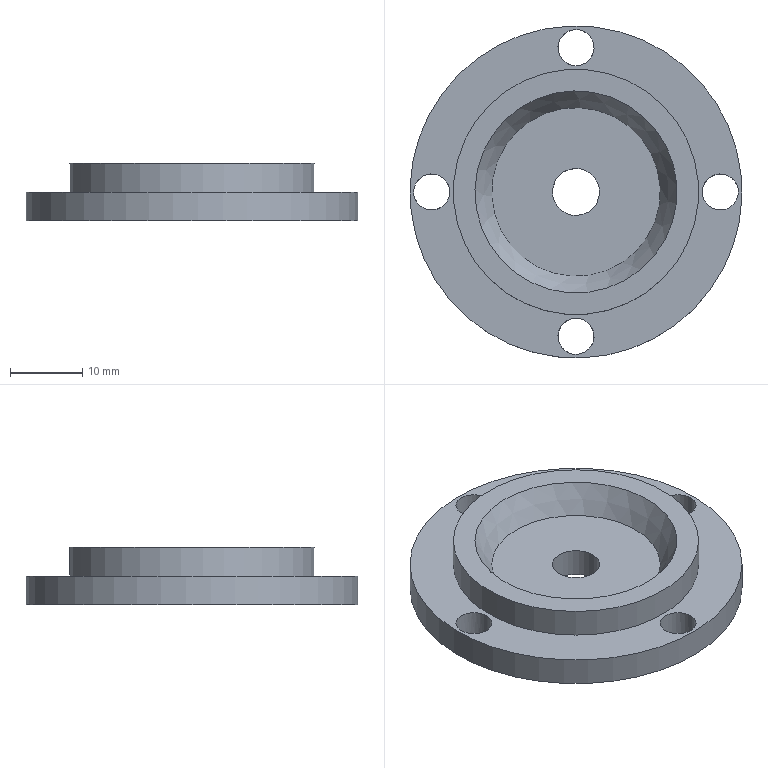Component | NX | BEARING_COVER | 1 solid | 12 faces | box 46 x 46 x 8 mm | volume 7753 mm3 | cylinder 7 | plane 4 | cone 1 | commonest cylinder face diameters 5 x4 46 x1 34 x1 6.5 x1
STEP:
#1=CARTESIAN_POINT('',(0.,0.,0.));
#2=DIRECTION('',(0.,0.,1.));
#3=DIRECTION('',(1.,0.,0.));
#4=AXIS2_PLACEMENT_3D('',#1,#2,#3);
#5=CARTESIAN_POINT('',(609.426,-134.038,-1192.));
#6=VERTEX_POINT('',#5);
#7=CARTESIAN_POINT('',(625.689,-150.302,-1192.));
#8=DIRECTION('',(0.,0.,1.));
#9=DIRECTION('',(-0.7071,0.7071,0.));
#10=AXIS2_PLACEMENT_3D('',#7,#8,#9);
#11=CIRCLE('',#10,23.);
#12=CARTESIAN_POINT('',(625.689,-150.302,-1188.));
#13=DIRECTION('',(0.,0.,1.));
#14=DIRECTION('',(-0.7071,0.7071,0.));
#15=AXIS2_PLACEMENT_3D('',#12,#13,#14);
#16=CYLINDRICAL_SURFACE('',#15,23.);
#17=CARTESIAN_POINT('',(0.,-4.));
#18=DIRECTION('',(1.,0.));
#19=VECTOR('',#18,1.);
#20=LINE('',#17,#19);
#21=(GEOMETRIC_REPRESENTATION_CONTEXT(2)PARAMETRIC_REPRESENTATION_CONTEXT()REPRESENTATION_CONTEXT('',''));
#22=DEFINITIONAL_REPRESENTATION('',(#20),#21);
#23=PCURVE('',#16,#22);
#24=CARTESIAN_POINT('',(641.952,-134.038,-1192.));
#25=DIRECTION('',(0.,0.,-1.));
#26=DIRECTION('',(0.7071,-0.7071,0.));
#27=AXIS2_PLACEMENT_3D('',#24,#25,#26);
#28=PLANE('',#27);
#29=CARTESIAN_POINT('',(-23.,23.));
#30=CARTESIAN_POINT('',(-23.,62.837));
#31=CARTESIAN_POINT('',(11.5,42.919));
#32=CARTESIAN_POINT('',(46.,23.));
#33=CARTESIAN_POINT('',(11.5,3.081));
#34=CARTESIAN_POINT('',(-23.,-16.837));
#35=CARTESIAN_POINT('',(-23.,23.));
#36=(BOUNDED_CURVE()B_SPLINE_CURVE(2,(#29,#30,#31,#32,#33,#34,#35),.UNSPECIFIED.,.T.,.F.)B_SPLINE_CURVE_WITH_KNOTS((1,2,2,2,2,1),(-2.094,0.,2.094,4.189,6.283,8.378),.UNSPECIFIED.)CURVE()GEOMETRIC_REPRESENTATION_ITEM()RATIONAL_B_SPLINE_CURVE((1.,0.5,1.,0.5,1.,0.5,1.))REPRESENTATION_ITEM(''));
#37=(GEOMETRIC_REPRESENTATION_CONTEXT(2)PARAMETRIC_REPRESENTATION_CONTEXT()REPRESENTATION_CONTEXT('',''));
#38=DEFINITIONAL_REPRESENTATION('',(#36),#37);
#39=PCURVE('',#28,#38);
#40=SURFACE_CURVE('',#11,(#23,#39),.PCURVE_S1.);
#41=EDGE_CURVE('',#6,#6,#40,.T.);
#42=ORIENTED_EDGE('',*,*,#41,.F.);
#43=CARTESIAN_POINT('',(609.426,-134.038,-1196.));
#44=VERTEX_POINT('',#43);
#45=CARTESIAN_POINT('',(609.426,-134.038,-1196.));
#46=CARTESIAN_POINT('',(609.426,-134.038,-1192.));
#47=B_SPLINE_CURVE_WITH_KNOTS('',1,(#45,#46),.UNSPECIFIED.,.F.,.F.,(2,2),(-8.,-4.),.PIECEWISE_BEZIER_KNOTS.);
#48=CARTESIAN_POINT('',(0.,0.));
#49=DIRECTION('',(0.,1.));
#50=VECTOR('',#49,1.);
#51=LINE('',#48,#50);
#52=(GEOMETRIC_REPRESENTATION_CONTEXT(2)PARAMETRIC_REPRESENTATION_CONTEXT()REPRESENTATION_CONTEXT('',''));
#53=DEFINITIONAL_REPRESENTATION('',(#51),#52);
#54=PCURVE('',#16,#53);
#55=CARTESIAN_POINT('',(6.283,0.));
#56=DIRECTION('',(0.,1.));
#57=VECTOR('',#56,1.);
#58=LINE('',#55,#57);
#59=(GEOMETRIC_REPRESENTATION_CONTEXT(2)PARAMETRIC_REPRESENTATION_CONTEXT()REPRESENTATION_CONTEXT('',''));
#60=DEFINITIONAL_REPRESENTATION('',(#58),#59);
#61=PCURVE('',#16,#60);
#62=SEAM_CURVE('',#47,(#54,#61),.PCURVE_S1.);
#63=EDGE_CURVE('',#44,#6,#62,.T.);
#64=ORIENTED_EDGE('',*,*,#63,.F.);
#65=CARTESIAN_POINT('',(625.689,-150.302,-1196.));
#66=DIRECTION('',(0.,0.,1.));
#67=DIRECTION('',(-0.7071,0.7071,0.));
#68=AXIS2_PLACEMENT_3D('',#65,#66,#67);
#69=CIRCLE('',#68,23.);
#70=CARTESIAN_POINT('',(0.,-8.));
#71=DIRECTION('',(1.,0.));
#72=VECTOR('',#71,1.);
#73=LINE('',#70,#72);
#74=(GEOMETRIC_REPRESENTATION_CONTEXT(2)PARAMETRIC_REPRESENTATION_CONTEXT()REPRESENTATION_CONTEXT('',''));
#75=DEFINITIONAL_REPRESENTATION('',(#73),#74);
#76=PCURVE('',#16,#75);
#77=CARTESIAN_POINT('',(627.987,-148.004,-1196.));
#78=DIRECTION('',(0.,0.,1.));
#79=DIRECTION('',(-0.7071,0.7071,0.));
#80=AXIS2_PLACEMENT_3D('',#77,#78,#79);
#81=PLANE('',#80);
#82=CARTESIAN_POINT('',(0.,3.25));
#83=DIRECTION('',(1.,0.));
#84=AXIS2_PLACEMENT_2D('',#82,#83);
#85=CIRCLE('',#84,23.);
#86=(GEOMETRIC_REPRESENTATION_CONTEXT(2)PARAMETRIC_REPRESENTATION_CONTEXT()REPRESENTATION_CONTEXT('',''));
#87=DEFINITIONAL_REPRESENTATION('',(#85),#86);
#88=PCURVE('',#81,#87);
#89=SURFACE_CURVE('',#69,(#76,#88),.PCURVE_S1.);
#90=EDGE_CURVE('',#44,#44,#89,.T.);
#91=ORIENTED_EDGE('',*,*,#90,.T.);
#92=ORIENTED_EDGE('',*,*,#63,.T.);
#93=EDGE_LOOP('',(#42,#64,#91,#92));
#94=FACE_BOUND('',#93,.T.);
#95=ADVANCED_FACE('',(#94),#16,.T.);
#96=CARTESIAN_POINT('',(627.457,-132.069,-1192.));
#97=VERTEX_POINT('',#96);
#98=CARTESIAN_POINT('',(625.689,-130.302,-1192.));
#99=DIRECTION('',(0.,0.,-1.));
#100=DIRECTION('',(0.7071,-0.7071,0.));
#101=AXIS2_PLACEMENT_3D('',#98,#99,#100);
#102=CIRCLE('',#101,2.5);
#103=CARTESIAN_POINT('',(-14.142,8.858));
#104=DIRECTION('',(1.,-0.));
#105=AXIS2_PLACEMENT_2D('',#103,#104);
#106=CIRCLE('',#105,2.5);
#107=(GEOMETRIC_REPRESENTATION_CONTEXT(2)PARAMETRIC_REPRESENTATION_CONTEXT()REPRESENTATION_CONTEXT('',''));
#108=DEFINITIONAL_REPRESENTATION('',(#106),#107);
#109=PCURVE('',#28,#108);
#110=CARTESIAN_POINT('',(625.689,-130.302,-1172.));
#111=DIRECTION('',(0.,0.,-1.));
#112=DIRECTION('',(0.7071,-0.7071,0.));
#113=AXIS2_PLACEMENT_3D('',#110,#111,#112);
#114=CYLINDRICAL_SURFACE('',#113,2.5);
#115=CARTESIAN_POINT('',(0.,20.));
#116=DIRECTION('',(1.,0.));
#117=VECTOR('',#116,1.);
#118=LINE('',#115,#117);
#119=(GEOMETRIC_REPRESENTATION_CONTEXT(2)PARAMETRIC_REPRESENTATION_CONTEXT()REPRESENTATION_CONTEXT('',''));
#120=DEFINITIONAL_REPRESENTATION('',(#118),#119);
#121=PCURVE('',#114,#120);
#122=SURFACE_CURVE('',#102,(#109,#121),.PCURVE_S1.);
#123=EDGE_CURVE('',#97,#97,#122,.T.);
#124=ORIENTED_EDGE('',*,*,#123,.T.);
#125=EDGE_LOOP('',(#124));
#126=FACE_BOUND('',#125,.T.);
#127=CARTESIAN_POINT('',(647.457,-152.069,-1192.));
#128=VERTEX_POINT('',#127);
#129=CARTESIAN_POINT('',(645.689,-150.302,-1192.));
#130=DIRECTION('',(0.,0.,-1.));
#131=DIRECTION('',(0.7071,-0.7071,0.));
#132=AXIS2_PLACEMENT_3D('',#129,#130,#131);
#133=CIRCLE('',#132,2.5);
#134=CARTESIAN_POINT('',(14.142,8.858));
#135=DIRECTION('',(1.,-0.));
#136=AXIS2_PLACEMENT_2D('',#134,#135);
#137=CIRCLE('',#136,2.5);
#138=(GEOMETRIC_REPRESENTATION_CONTEXT(2)PARAMETRIC_REPRESENTATION_CONTEXT()REPRESENTATION_CONTEXT('',''));
#139=DEFINITIONAL_REPRESENTATION('',(#137),#138);
#140=PCURVE('',#28,#139);
#141=CARTESIAN_POINT('',(645.689,-150.302,-1172.));
#142=DIRECTION('',(0.,0.,-1.));
#143=DIRECTION('',(0.7071,-0.7071,0.));
#144=AXIS2_PLACEMENT_3D('',#141,#142,#143);
#145=CYLINDRICAL_SURFACE('',#144,2.5);
#146=CARTESIAN_POINT('',(0.,20.));
#147=DIRECTION('',(1.,0.));
#148=VECTOR('',#147,1.);
#149=LINE('',#146,#148);
#150=(GEOMETRIC_REPRESENTATION_CONTEXT(2)PARAMETRIC_REPRESENTATION_CONTEXT()REPRESENTATION_CONTEXT('',''));
#151=DEFINITIONAL_REPRESENTATION('',(#149),#150);
#152=PCURVE('',#145,#151);
#153=SURFACE_CURVE('',#133,(#140,#152),.PCURVE_S1.);
#154=EDGE_CURVE('',#128,#128,#153,.T.);
#155=ORIENTED_EDGE('',*,*,#154,.T.);
#156=EDGE_LOOP('',(#155));
#157=FACE_BOUND('',#156,.T.);
#158=CARTESIAN_POINT('',(607.457,-152.069,-1192.));
#159=VERTEX_POINT('',#158);
#160=CARTESIAN_POINT('',(605.689,-150.302,-1192.));
#161=DIRECTION('',(0.,0.,-1.));
#162=DIRECTION('',(0.7071,-0.7071,0.));
#163=AXIS2_PLACEMENT_3D('',#160,#161,#162);
#164=CIRCLE('',#163,2.5);
#165=CARTESIAN_POINT('',(-14.142,37.142));
#166=DIRECTION('',(1.,-0.));
#167=AXIS2_PLACEMENT_2D('',#165,#166);
#168=CIRCLE('',#167,2.5);
#169=(GEOMETRIC_REPRESENTATION_CONTEXT(2)PARAMETRIC_REPRESENTATION_CONTEXT()REPRESENTATION_CONTEXT('',''));
#170=DEFINITIONAL_REPRESENTATION('',(#168),#169);
#171=PCURVE('',#28,#170);
#172=CARTESIAN_POINT('',(605.689,-150.302,-1172.));
#173=DIRECTION('',(0.,0.,-1.));
#174=DIRECTION('',(0.7071,-0.7071,0.));
#175=AXIS2_PLACEMENT_3D('',#172,#173,#174);
#176=CYLINDRICAL_SURFACE('',#175,2.5);
#177=CARTESIAN_POINT('',(0.,20.));
#178=DIRECTION('',(1.,0.));
#179=VECTOR('',#178,1.);
#180=LINE('',#177,#179);
#181=(GEOMETRIC_REPRESENTATION_CONTEXT(2)PARAMETRIC_REPRESENTATION_CONTEXT()REPRESENTATION_CONTEXT('',''));
#182=DEFINITIONAL_REPRESENTATION('',(#180),#181);
#183=PCURVE('',#176,#182);
#184=SURFACE_CURVE('',#164,(#171,#183),.PCURVE_S1.);
#185=EDGE_CURVE('',#159,#159,#184,.T.);
#186=ORIENTED_EDGE('',*,*,#185,.T.);
#187=EDGE_LOOP('',(#186));
#188=FACE_BOUND('',#187,.T.);
#189=CARTESIAN_POINT('',(627.457,-172.069,-1192.));
#190=VERTEX_POINT('',#189);
#191=CARTESIAN_POINT('',(625.689,-170.302,-1192.));
#192=DIRECTION('',(0.,0.,-1.));
#193=DIRECTION('',(0.7071,-0.7071,0.));
#194=AXIS2_PLACEMENT_3D('',#191,#192,#193);
#195=CIRCLE('',#194,2.5);
#196=CARTESIAN_POINT('',(14.142,37.142));
#197=DIRECTION('',(1.,-0.));
#198=AXIS2_PLACEMENT_2D('',#196,#197);
#199=CIRCLE('',#198,2.5);
#200=(GEOMETRIC_REPRESENTATION_CONTEXT(2)PARAMETRIC_REPRESENTATION_CONTEXT()REPRESENTATION_CONTEXT('',''));
#201=DEFINITIONAL_REPRESENTATION('',(#199),#200);
#202=PCURVE('',#28,#201);
#203=CARTESIAN_POINT('',(625.689,-170.302,-1172.));
#204=DIRECTION('',(0.,0.,-1.));
#205=DIRECTION('',(0.7071,-0.7071,0.));
#206=AXIS2_PLACEMENT_3D('',#203,#204,#205);
#207=CYLINDRICAL_SURFACE('',#206,2.5);
#208=CARTESIAN_POINT('',(0.,20.));
#209=DIRECTION('',(1.,0.));
#210=VECTOR('',#209,1.);
#211=LINE('',#208,#210);
#212=(GEOMETRIC_REPRESENTATION_CONTEXT(2)PARAMETRIC_REPRESENTATION_CONTEXT()REPRESENTATION_CONTEXT('',''));
#213=DEFINITIONAL_REPRESENTATION('',(#211),#212);
#214=PCURVE('',#207,#213);
#215=SURFACE_CURVE('',#195,(#202,#214),.PCURVE_S1.);
#216=EDGE_CURVE('',#190,#190,#215,.T.);
#217=ORIENTED_EDGE('',*,*,#216,.T.);
#218=EDGE_LOOP('',(#217));
#219=FACE_BOUND('',#218,.T.);
#220=CARTESIAN_POINT('',(613.668,-138.281,-1192.));
#221=VERTEX_POINT('',#220);
#222=CARTESIAN_POINT('',(625.689,-150.302,-1192.));
#223=DIRECTION('',(0.,0.,1.));
#224=DIRECTION('',(-0.7071,0.7071,0.));
#225=AXIS2_PLACEMENT_3D('',#222,#223,#224);
#226=CIRCLE('',#225,17.);
#227=CARTESIAN_POINT('',(-17.,23.));
#228=CARTESIAN_POINT('',(-17.,52.445));
#229=CARTESIAN_POINT('',(8.5,37.722));
#230=CARTESIAN_POINT('',(34.,23.));
#231=CARTESIAN_POINT('',(8.5,8.278));
#232=CARTESIAN_POINT('',(-17.,-6.445));
#233=CARTESIAN_POINT('',(-17.,23.));
#234=(BOUNDED_CURVE()B_SPLINE_CURVE(2,(#227,#228,#229,#230,#231,#232,#233),.UNSPECIFIED.,.T.,.F.)B_SPLINE_CURVE_WITH_KNOTS((1,2,2,2,2,1),(-2.094,0.,2.094,4.189,6.283,8.378),.UNSPECIFIED.)CURVE()GEOMETRIC_REPRESENTATION_ITEM()RATIONAL_B_SPLINE_CURVE((1.,0.5,1.,0.5,1.,0.5,1.))REPRESENTATION_ITEM(''));
#235=(GEOMETRIC_REPRESENTATION_CONTEXT(2)PARAMETRIC_REPRESENTATION_CONTEXT()REPRESENTATION_CONTEXT('',''));
#236=DEFINITIONAL_REPRESENTATION('',(#234),#235);
#237=PCURVE('',#28,#236);
#238=CARTESIAN_POINT('',(625.689,-150.302,-1188.));
#239=DIRECTION('',(0.,0.,1.));
#240=DIRECTION('',(-0.7071,0.7071,0.));
#241=AXIS2_PLACEMENT_3D('',#238,#239,#240);
#242=CYLINDRICAL_SURFACE('',#241,17.);
#243=CARTESIAN_POINT('',(0.,-4.));
#244=DIRECTION('',(1.,0.));
#245=VECTOR('',#244,1.);
#246=LINE('',#243,#245);
#247=(GEOMETRIC_REPRESENTATION_CONTEXT(2)PARAMETRIC_REPRESENTATION_CONTEXT()REPRESENTATION_CONTEXT('',''));
#248=DEFINITIONAL_REPRESENTATION('',(#246),#247);
#249=PCURVE('',#242,#248);
#250=SURFACE_CURVE('',#226,(#237,#249),.PCURVE_S1.);
#251=EDGE_CURVE('',#221,#221,#250,.T.);
#252=ORIENTED_EDGE('',*,*,#251,.F.);
#253=EDGE_LOOP('',(#252));
#254=FACE_BOUND('',#253,.T.);
#255=ORIENTED_EDGE('',*,*,#41,.T.);
#256=EDGE_LOOP('',(#255));
#257=FACE_BOUND('',#256,.T.);
#258=ADVANCED_FACE('',(#126,#157,#188,#219,#254,#257),#28,.F.);
#259=CARTESIAN_POINT('',(613.668,-138.281,-1188.));
#260=VERTEX_POINT('',#259);
#261=CARTESIAN_POINT('',(625.689,-150.302,-1188.));
#262=DIRECTION('',(0.,0.,1.));
#263=DIRECTION('',(-0.7071,0.7071,0.));
#264=AXIS2_PLACEMENT_3D('',#261,#262,#263);
#265=CIRCLE('',#264,17.);
#266=CARTESIAN_POINT('',(0.,0.));
#267=DIRECTION('',(1.,0.));
#268=VECTOR('',#267,1.);
#269=LINE('',#266,#268);
#270=(GEOMETRIC_REPRESENTATION_CONTEXT(2)PARAMETRIC_REPRESENTATION_CONTEXT()REPRESENTATION_CONTEXT('',''));
#271=DEFINITIONAL_REPRESENTATION('',(#269),#270);
#272=PCURVE('',#242,#271);
#273=CARTESIAN_POINT('',(637.71,-138.281,-1188.));
#274=DIRECTION('',(0.,0.,-1.));
#275=DIRECTION('',(0.7071,-0.7071,0.));
#276=AXIS2_PLACEMENT_3D('',#273,#274,#275);
#277=PLANE('',#276);
#278=CARTESIAN_POINT('',(-17.,17.));
#279=CARTESIAN_POINT('',(-17.,46.445));
#280=CARTESIAN_POINT('',(8.5,31.722));
#281=CARTESIAN_POINT('',(34.,17.));
#282=CARTESIAN_POINT('',(8.5,2.278));
#283=CARTESIAN_POINT('',(-17.,-12.445));
#284=CARTESIAN_POINT('',(-17.,17.));
#285=(BOUNDED_CURVE()B_SPLINE_CURVE(2,(#278,#279,#280,#281,#282,#283,#284),.UNSPECIFIED.,.T.,.F.)B_SPLINE_CURVE_WITH_KNOTS((1,2,2,2,2,1),(-2.094,0.,2.094,4.189,6.283,8.378),.UNSPECIFIED.)CURVE()GEOMETRIC_REPRESENTATION_ITEM()RATIONAL_B_SPLINE_CURVE((1.,0.5,1.,0.5,1.,0.5,1.))REPRESENTATION_ITEM(''));
#286=(GEOMETRIC_REPRESENTATION_CONTEXT(2)PARAMETRIC_REPRESENTATION_CONTEXT()REPRESENTATION_CONTEXT('',''));
#287=DEFINITIONAL_REPRESENTATION('',(#285),#286);
#288=PCURVE('',#277,#287);
#289=SURFACE_CURVE('',#265,(#272,#288),.PCURVE_S1.);
#290=EDGE_CURVE('',#260,#260,#289,.T.);
#291=ORIENTED_EDGE('',*,*,#290,.F.);
#292=CARTESIAN_POINT('',(613.668,-138.281,-1192.));
#293=CARTESIAN_POINT('',(613.668,-138.281,-1188.));
#294=B_SPLINE_CURVE_WITH_KNOTS('',1,(#292,#293),.UNSPECIFIED.,.F.,.F.,(2,2),(-4.,0.),.PIECEWISE_BEZIER_KNOTS.);
#295=CARTESIAN_POINT('',(0.,0.));
#296=DIRECTION('',(0.,1.));
#297=VECTOR('',#296,1.);
#298=LINE('',#295,#297);
#299=(GEOMETRIC_REPRESENTATION_CONTEXT(2)PARAMETRIC_REPRESENTATION_CONTEXT()REPRESENTATION_CONTEXT('',''));
#300=DEFINITIONAL_REPRESENTATION('',(#298),#299);
#301=PCURVE('',#242,#300);
#302=CARTESIAN_POINT('',(6.283,0.));
#303=DIRECTION('',(0.,1.));
#304=VECTOR('',#303,1.);
#305=LINE('',#302,#304);
#306=(GEOMETRIC_REPRESENTATION_CONTEXT(2)PARAMETRIC_REPRESENTATION_CONTEXT()REPRESENTATION_CONTEXT('',''));
#307=DEFINITIONAL_REPRESENTATION('',(#305),#306);
#308=PCURVE('',#242,#307);
#309=SEAM_CURVE('',#294,(#301,#308),.PCURVE_S1.);
#310=EDGE_CURVE('',#221,#260,#309,.T.);
#311=ORIENTED_EDGE('',*,*,#310,.F.);
#312=ORIENTED_EDGE('',*,*,#251,.T.);
#313=ORIENTED_EDGE('',*,*,#310,.T.);
#314=EDGE_LOOP('',(#291,#311,#312,#313));
#315=FACE_BOUND('',#314,.T.);
#316=ADVANCED_FACE('',(#315),#242,.T.);
#317=CARTESIAN_POINT('',(615.79,-140.402,-1188.));
#318=VERTEX_POINT('',#317);
#319=CARTESIAN_POINT('',(625.689,-150.302,-1188.));
#320=DIRECTION('',(0.,0.,1.));
#321=DIRECTION('',(-0.7071,0.7071,0.));
#322=AXIS2_PLACEMENT_3D('',#319,#320,#321);
#323=CIRCLE('',#322,14.);
#324=CARTESIAN_POINT('',(-14.,17.));
#325=CARTESIAN_POINT('',(-14.,41.249));
#326=CARTESIAN_POINT('',(7.,29.124));
#327=CARTESIAN_POINT('',(28.,17.));
#328=CARTESIAN_POINT('',(7.,4.876));
#329=CARTESIAN_POINT('',(-14.,-7.249));
#330=CARTESIAN_POINT('',(-14.,17.));
#331=(BOUNDED_CURVE()B_SPLINE_CURVE(2,(#324,#325,#326,#327,#328,#329,#330),.UNSPECIFIED.,.T.,.F.)B_SPLINE_CURVE_WITH_KNOTS((1,2,2,2,2,1),(-2.094,0.,2.094,4.189,6.283,8.378),.UNSPECIFIED.)CURVE()GEOMETRIC_REPRESENTATION_ITEM()RATIONAL_B_SPLINE_CURVE((1.,0.5,1.,0.5,1.,0.5,1.))REPRESENTATION_ITEM(''));
#332=(GEOMETRIC_REPRESENTATION_CONTEXT(2)PARAMETRIC_REPRESENTATION_CONTEXT()REPRESENTATION_CONTEXT('',''));
#333=DEFINITIONAL_REPRESENTATION('',(#331),#332);
#334=PCURVE('',#277,#333);
#335=CARTESIAN_POINT('',(625.689,-150.302,-1188.));
#336=DIRECTION('',(0.,0.,1.));
#337=DIRECTION('',(-0.7071,0.7071,0.));
#338=AXIS2_PLACEMENT_3D('',#335,#336,#337);
#339=CONICAL_SURFACE('',#338,14.,0.5236);
#340=CARTESIAN_POINT('',(0.,-0.));
#341=DIRECTION('',(1.,0.));
#342=VECTOR('',#341,1.);
#343=LINE('',#340,#342);
#344=(GEOMETRIC_REPRESENTATION_CONTEXT(2)PARAMETRIC_REPRESENTATION_CONTEXT()REPRESENTATION_CONTEXT('',''));
#345=DEFINITIONAL_REPRESENTATION('',(#343),#344);
#346=PCURVE('',#339,#345);
#347=SURFACE_CURVE('',#323,(#334,#346),.PCURVE_S1.);
#348=EDGE_CURVE('',#318,#318,#347,.T.);
#349=ORIENTED_EDGE('',*,*,#348,.F.);
#350=EDGE_LOOP('',(#349));
#351=FACE_BOUND('',#350,.T.);
#352=ORIENTED_EDGE('',*,*,#290,.T.);
#353=EDGE_LOOP('',(#352));
#354=FACE_BOUND('',#353,.T.);
#355=ADVANCED_FACE('',(#351,#354),#277,.F.);
#356=CARTESIAN_POINT('',(617.422,-142.035,-1192.));
#357=VERTEX_POINT('',#356);
#358=CARTESIAN_POINT('',(625.689,-150.302,-1192.));
#359=DIRECTION('',(0.,0.,1.));
#360=DIRECTION('',(-0.7071,0.7071,0.));
#361=AXIS2_PLACEMENT_3D('',#358,#359,#360);
#362=CIRCLE('',#361,11.691);
#363=CARTESIAN_POINT('',(0.,-4.));
#364=DIRECTION('',(1.,0.));
#365=VECTOR('',#364,1.);
#366=LINE('',#363,#365);
#367=(GEOMETRIC_REPRESENTATION_CONTEXT(2)PARAMETRIC_REPRESENTATION_CONTEXT()REPRESENTATION_CONTEXT('',''));
#368=DEFINITIONAL_REPRESENTATION('',(#366),#367);
#369=PCURVE('',#339,#368);
#370=CARTESIAN_POINT('',(633.956,-142.035,-1192.));
#371=DIRECTION('',(0.,0.,-1.));
#372=DIRECTION('',(0.7071,-0.7071,0.));
#373=AXIS2_PLACEMENT_3D('',#370,#371,#372);
#374=PLANE('',#373);
#375=CARTESIAN_POINT('',(-11.691,11.691));
#376=CARTESIAN_POINT('',(-11.691,31.939));
#377=CARTESIAN_POINT('',(5.845,21.815));
#378=CARTESIAN_POINT('',(23.381,11.691));
#379=CARTESIAN_POINT('',(5.845,1.566));
#380=CARTESIAN_POINT('',(-11.691,-8.558));
#381=CARTESIAN_POINT('',(-11.691,11.691));
#382=(BOUNDED_CURVE()B_SPLINE_CURVE(2,(#375,#376,#377,#378,#379,#380,#381),.UNSPECIFIED.,.T.,.F.)B_SPLINE_CURVE_WITH_KNOTS((1,2,2,2,2,1),(-2.094,0.,2.094,4.189,6.283,8.378),.UNSPECIFIED.)CURVE()GEOMETRIC_REPRESENTATION_ITEM()RATIONAL_B_SPLINE_CURVE((1.,0.5,1.,0.5,1.,0.5,1.))REPRESENTATION_ITEM(''));
#383=(GEOMETRIC_REPRESENTATION_CONTEXT(2)PARAMETRIC_REPRESENTATION_CONTEXT()REPRESENTATION_CONTEXT('',''));
#384=DEFINITIONAL_REPRESENTATION('',(#382),#383);
#385=PCURVE('',#374,#384);
#386=SURFACE_CURVE('',#362,(#369,#385),.PCURVE_S1.);
#387=EDGE_CURVE('',#357,#357,#386,.T.);
#388=ORIENTED_EDGE('',*,*,#387,.T.);
#389=CARTESIAN_POINT('',(617.422,-142.035,-1192.));
#390=CARTESIAN_POINT('',(615.79,-140.402,-1188.));
#391=B_SPLINE_CURVE_WITH_KNOTS('',1,(#389,#390),.UNSPECIFIED.,.F.,.F.,(2,2),(-4.619,-0.),.PIECEWISE_BEZIER_KNOTS.);
#392=CARTESIAN_POINT('',(6.283,0.));
#393=DIRECTION('',(0.,1.));
#394=VECTOR('',#393,1.);
#395=LINE('',#392,#394);
#396=(GEOMETRIC_REPRESENTATION_CONTEXT(2)PARAMETRIC_REPRESENTATION_CONTEXT()REPRESENTATION_CONTEXT('',''));
#397=DEFINITIONAL_REPRESENTATION('',(#395),#396);
#398=PCURVE('',#339,#397);
#399=CARTESIAN_POINT('',(0.,0.));
#400=DIRECTION('',(0.,1.));
#401=VECTOR('',#400,1.);
#402=LINE('',#399,#401);
#403=(GEOMETRIC_REPRESENTATION_CONTEXT(2)PARAMETRIC_REPRESENTATION_CONTEXT()REPRESENTATION_CONTEXT('',''));
#404=DEFINITIONAL_REPRESENTATION('',(#402),#403);
#405=PCURVE('',#339,#404);
#406=SEAM_CURVE('',#391,(#398,#405),.PCURVE_S1.);
#407=EDGE_CURVE('',#357,#318,#406,.T.);
#408=ORIENTED_EDGE('',*,*,#407,.T.);
#409=ORIENTED_EDGE('',*,*,#348,.F.);
#410=ORIENTED_EDGE('',*,*,#407,.F.);
#411=EDGE_LOOP('',(#388,#408,#409,#410));
#412=FACE_BOUND('',#411,.F.);
#413=ADVANCED_FACE('',(#412),#339,.F.);
#414=CARTESIAN_POINT('',(623.391,-148.004,-1192.));
#415=VERTEX_POINT('',#414);
#416=CARTESIAN_POINT('',(625.689,-150.302,-1192.));
#417=DIRECTION('',(0.,0.,1.));
#418=DIRECTION('',(-0.7071,0.7071,0.));
#419=AXIS2_PLACEMENT_3D('',#416,#417,#418);
#420=CIRCLE('',#419,3.25);
#421=CARTESIAN_POINT('',(-3.25,11.691));
#422=CARTESIAN_POINT('',(-3.25,17.32));
#423=CARTESIAN_POINT('',(1.625,14.505));
#424=CARTESIAN_POINT('',(6.5,11.691));
#425=CARTESIAN_POINT('',(1.625,8.876));
#426=CARTESIAN_POINT('',(-3.25,6.061));
#427=CARTESIAN_POINT('',(-3.25,11.691));
#428=(BOUNDED_CURVE()B_SPLINE_CURVE(2,(#421,#422,#423,#424,#425,#426,#427),.UNSPECIFIED.,.T.,.F.)B_SPLINE_CURVE_WITH_KNOTS((1,2,2,2,2,1),(-2.094,0.,2.094,4.189,6.283,8.378),.UNSPECIFIED.)CURVE()GEOMETRIC_REPRESENTATION_ITEM()RATIONAL_B_SPLINE_CURVE((1.,0.5,1.,0.5,1.,0.5,1.))REPRESENTATION_ITEM(''));
#429=(GEOMETRIC_REPRESENTATION_CONTEXT(2)PARAMETRIC_REPRESENTATION_CONTEXT()REPRESENTATION_CONTEXT('',''));
#430=DEFINITIONAL_REPRESENTATION('',(#428),#429);
#431=PCURVE('',#374,#430);
#432=CARTESIAN_POINT('',(625.689,-150.302,-1188.));
#433=DIRECTION('',(0.,0.,1.));
#434=DIRECTION('',(-0.7071,0.7071,0.));
#435=AXIS2_PLACEMENT_3D('',#432,#433,#434);
#436=CYLINDRICAL_SURFACE('',#435,3.25);
#437=CARTESIAN_POINT('',(0.,-4.));
#438=DIRECTION('',(1.,0.));
#439=VECTOR('',#438,1.);
#440=LINE('',#437,#439);
#441=(GEOMETRIC_REPRESENTATION_CONTEXT(2)PARAMETRIC_REPRESENTATION_CONTEXT()REPRESENTATION_CONTEXT('',''));
#442=DEFINITIONAL_REPRESENTATION('',(#440),#441);
#443=PCURVE('',#436,#442);
#444=SURFACE_CURVE('',#420,(#431,#443),.PCURVE_S1.);
#445=EDGE_CURVE('',#415,#415,#444,.T.);
#446=ORIENTED_EDGE('',*,*,#445,.F.);
#447=EDGE_LOOP('',(#446));
#448=FACE_BOUND('',#447,.T.);
#449=ORIENTED_EDGE('',*,*,#387,.T.);
#450=EDGE_LOOP('',(#449));
#451=FACE_BOUND('',#450,.T.);
#452=ADVANCED_FACE('',(#448,#451),#374,.F.);
#453=CARTESIAN_POINT('',(623.391,-148.004,-1196.));
#454=VERTEX_POINT('',#453);
#455=CARTESIAN_POINT('',(625.689,-150.302,-1196.));
#456=DIRECTION('',(0.,0.,1.));
#457=DIRECTION('',(-0.7071,0.7071,0.));
#458=AXIS2_PLACEMENT_3D('',#455,#456,#457);
#459=CIRCLE('',#458,3.25);
#460=CARTESIAN_POINT('',(0.,-8.));
#461=DIRECTION('',(1.,0.));
#462=VECTOR('',#461,1.);
#463=LINE('',#460,#462);
#464=(GEOMETRIC_REPRESENTATION_CONTEXT(2)PARAMETRIC_REPRESENTATION_CONTEXT()REPRESENTATION_CONTEXT('',''));
#465=DEFINITIONAL_REPRESENTATION('',(#463),#464);
#466=PCURVE('',#436,#465);
#467=CARTESIAN_POINT('',(0.,3.25));
#468=DIRECTION('',(1.,0.));
#469=AXIS2_PLACEMENT_2D('',#467,#468);
#470=CIRCLE('',#469,3.25);
#471=(GEOMETRIC_REPRESENTATION_CONTEXT(2)PARAMETRIC_REPRESENTATION_CONTEXT()REPRESENTATION_CONTEXT('',''));
#472=DEFINITIONAL_REPRESENTATION('',(#470),#471);
#473=PCURVE('',#81,#472);
#474=SURFACE_CURVE('',#459,(#466,#473),.PCURVE_S1.);
#475=EDGE_CURVE('',#454,#454,#474,.T.);
#476=ORIENTED_EDGE('',*,*,#475,.T.);
#477=CARTESIAN_POINT('',(623.391,-148.004,-1196.));
#478=CARTESIAN_POINT('',(623.391,-148.004,-1192.));
#479=B_SPLINE_CURVE_WITH_KNOTS('',1,(#477,#478),.UNSPECIFIED.,.F.,.F.,(2,2),(-8.,-4.),.PIECEWISE_BEZIER_KNOTS.);
#480=CARTESIAN_POINT('',(6.283,0.));
#481=DIRECTION('',(0.,1.));
#482=VECTOR('',#481,1.);
#483=LINE('',#480,#482);
#484=(GEOMETRIC_REPRESENTATION_CONTEXT(2)PARAMETRIC_REPRESENTATION_CONTEXT()REPRESENTATION_CONTEXT('',''));
#485=DEFINITIONAL_REPRESENTATION('',(#483),#484);
#486=PCURVE('',#436,#485);
#487=CARTESIAN_POINT('',(0.,0.));
#488=DIRECTION('',(0.,1.));
#489=VECTOR('',#488,1.);
#490=LINE('',#487,#489);
#491=(GEOMETRIC_REPRESENTATION_CONTEXT(2)PARAMETRIC_REPRESENTATION_CONTEXT()REPRESENTATION_CONTEXT('',''));
#492=DEFINITIONAL_REPRESENTATION('',(#490),#491);
#493=PCURVE('',#436,#492);
#494=SEAM_CURVE('',#479,(#486,#493),.PCURVE_S1.);
#495=EDGE_CURVE('',#454,#415,#494,.T.);
#496=ORIENTED_EDGE('',*,*,#495,.T.);
#497=ORIENTED_EDGE('',*,*,#445,.F.);
#498=ORIENTED_EDGE('',*,*,#495,.F.);
#499=EDGE_LOOP('',(#476,#496,#497,#498));
#500=FACE_BOUND('',#499,.F.);
#501=ADVANCED_FACE('',(#500),#436,.F.);
#502=CARTESIAN_POINT('',(625.689,-132.802,-1196.));
#503=VERTEX_POINT('',#502);
#504=CARTESIAN_POINT('',(627.457,-132.069,-1196.));
#505=VERTEX_POINT('',#504);
#506=CARTESIAN_POINT('',(625.689,-130.302,-1196.));
#507=DIRECTION('',(0.,0.,-1.));
#508=DIRECTION('',(0.,-1.,0.));
#509=AXIS2_PLACEMENT_3D('',#506,#507,#508);
#510=CIRCLE('',#509,2.5);
#511=CARTESIAN_POINT('',(12.374,-9.124));
#512=CARTESIAN_POINT('',(15.436,-6.063));
#513=CARTESIAN_POINT('',(16.557,-10.245));
#514=CARTESIAN_POINT('',(17.678,-14.428));
#515=CARTESIAN_POINT('',(13.495,-13.307));
#516=CARTESIAN_POINT('',(9.313,-12.186));
#517=CARTESIAN_POINT('',(12.374,-9.124));
#518=(BOUNDED_CURVE()B_SPLINE_CURVE(2,(#511,#512,#513,#514,#515,#516,#517),.UNSPECIFIED.,.T.,.F.)B_SPLINE_CURVE_WITH_KNOTS((1,2,2,2,2,1),(-2.094,0.,2.094,4.189,6.283,8.378),.UNSPECIFIED.)CURVE()GEOMETRIC_REPRESENTATION_ITEM()RATIONAL_B_SPLINE_CURVE((1.,0.5,1.,0.5,1.,0.5,1.))REPRESENTATION_ITEM(''));
#519=(GEOMETRIC_REPRESENTATION_CONTEXT(2)PARAMETRIC_REPRESENTATION_CONTEXT()REPRESENTATION_CONTEXT('',''));
#520=DEFINITIONAL_REPRESENTATION('',(#518),#519);
#521=PCURVE('',#81,#520);
#522=CARTESIAN_POINT('',(0.7854,24.));
#523=DIRECTION('',(1.,0.));
#524=VECTOR('',#523,1.);
#525=LINE('',#522,#524);
#526=(GEOMETRIC_REPRESENTATION_CONTEXT(2)PARAMETRIC_REPRESENTATION_CONTEXT()REPRESENTATION_CONTEXT('',''));
#527=DEFINITIONAL_REPRESENTATION('',(#525),#526);
#528=PCURVE('',#114,#527);
#529=SURFACE_CURVE('',#510,(#521,#528),.PCURVE_S1.);
#530=EDGE_CURVE('',#503,#505,#529,.T.);
#531=ORIENTED_EDGE('',*,*,#530,.F.);
#532=CARTESIAN_POINT('',(625.689,-130.302,-1196.));
#533=DIRECTION('',(0.,0.,-1.));
#534=DIRECTION('',(0.,-1.,0.));
#535=AXIS2_PLACEMENT_3D('',#532,#533,#534);
#536=CIRCLE('',#535,2.5);
#537=CARTESIAN_POINT('',(12.374,-9.124));
#538=CARTESIAN_POINT('',(15.436,-6.063));
#539=CARTESIAN_POINT('',(16.557,-10.245));
#540=CARTESIAN_POINT('',(17.678,-14.428));
#541=CARTESIAN_POINT('',(13.495,-13.307));
#542=CARTESIAN_POINT('',(9.313,-12.186));
#543=CARTESIAN_POINT('',(12.374,-9.124));
#544=(BOUNDED_CURVE()B_SPLINE_CURVE(2,(#537,#538,#539,#540,#541,#542,#543),.UNSPECIFIED.,.T.,.F.)B_SPLINE_CURVE_WITH_KNOTS((1,2,2,2,2,1),(-2.094,0.,2.094,4.189,6.283,8.378),.UNSPECIFIED.)CURVE()GEOMETRIC_REPRESENTATION_ITEM()RATIONAL_B_SPLINE_CURVE((1.,0.5,1.,0.5,1.,0.5,1.))REPRESENTATION_ITEM(''));
#545=(GEOMETRIC_REPRESENTATION_CONTEXT(2)PARAMETRIC_REPRESENTATION_CONTEXT()REPRESENTATION_CONTEXT('',''));
#546=DEFINITIONAL_REPRESENTATION('',(#544),#545);
#547=PCURVE('',#81,#546);
#548=CARTESIAN_POINT('',(-5.498,24.));
#549=DIRECTION('',(1.,0.));
#550=VECTOR('',#549,1.);
#551=LINE('',#548,#550);
#552=(GEOMETRIC_REPRESENTATION_CONTEXT(2)PARAMETRIC_REPRESENTATION_CONTEXT()REPRESENTATION_CONTEXT('',''));
#553=DEFINITIONAL_REPRESENTATION('',(#551),#552);
#554=PCURVE('',#114,#553);
#555=SURFACE_CURVE('',#536,(#547,#554),.PCURVE_S1.);
#556=EDGE_CURVE('',#505,#503,#555,.T.);
#557=ORIENTED_EDGE('',*,*,#556,.F.);
#558=EDGE_LOOP('',(#531,#557));
#559=FACE_BOUND('',#558,.T.);
#560=CARTESIAN_POINT('',(643.189,-150.302,-1196.));
#561=VERTEX_POINT('',#560);
#562=CARTESIAN_POINT('',(647.457,-152.069,-1196.));
#563=VERTEX_POINT('',#562);
#564=CARTESIAN_POINT('',(645.689,-150.302,-1196.));
#565=DIRECTION('',(0.,0.,-1.));
#566=DIRECTION('',(-1.,-0.,0.));
#567=AXIS2_PLACEMENT_3D('',#564,#565,#566);
#568=CIRCLE('',#567,2.5);
#569=CARTESIAN_POINT('',(-12.374,-9.124));
#570=CARTESIAN_POINT('',(-9.313,-12.186));
#571=CARTESIAN_POINT('',(-13.495,-13.307));
#572=CARTESIAN_POINT('',(-17.678,-14.428));
#573=CARTESIAN_POINT('',(-16.557,-10.245));
#574=CARTESIAN_POINT('',(-15.436,-6.063));
#575=CARTESIAN_POINT('',(-12.374,-9.124));
#576=(BOUNDED_CURVE()B_SPLINE_CURVE(2,(#569,#570,#571,#572,#573,#574,#575),.UNSPECIFIED.,.T.,.F.)B_SPLINE_CURVE_WITH_KNOTS((1,2,2,2,2,1),(-2.094,0.,2.094,4.189,6.283,8.378),.UNSPECIFIED.)CURVE()GEOMETRIC_REPRESENTATION_ITEM()RATIONAL_B_SPLINE_CURVE((1.,0.5,1.,0.5,1.,0.5,1.))REPRESENTATION_ITEM(''));
#577=(GEOMETRIC_REPRESENTATION_CONTEXT(2)PARAMETRIC_REPRESENTATION_CONTEXT()REPRESENTATION_CONTEXT('',''));
#578=DEFINITIONAL_REPRESENTATION('',(#576),#577);
#579=PCURVE('',#81,#578);
#580=CARTESIAN_POINT('',(2.356,24.));
#581=DIRECTION('',(1.,0.));
#582=VECTOR('',#581,1.);
#583=LINE('',#580,#582);
#584=(GEOMETRIC_REPRESENTATION_CONTEXT(2)PARAMETRIC_REPRESENTATION_CONTEXT()REPRESENTATION_CONTEXT('',''));
#585=DEFINITIONAL_REPRESENTATION('',(#583),#584);
#586=PCURVE('',#145,#585);
#587=SURFACE_CURVE('',#568,(#579,#586),.PCURVE_S1.);
#588=EDGE_CURVE('',#561,#563,#587,.T.);
#589=ORIENTED_EDGE('',*,*,#588,.F.);
#590=CARTESIAN_POINT('',(645.689,-150.302,-1196.));
#591=DIRECTION('',(0.,0.,-1.));
#592=DIRECTION('',(-1.,-0.,0.));
#593=AXIS2_PLACEMENT_3D('',#590,#591,#592);
#594=CIRCLE('',#593,2.5);
#595=CARTESIAN_POINT('',(-12.374,-9.124));
#596=CARTESIAN_POINT('',(-9.313,-12.186));
#597=CARTESIAN_POINT('',(-13.495,-13.307));
#598=CARTESIAN_POINT('',(-17.678,-14.428));
#599=CARTESIAN_POINT('',(-16.557,-10.245));
#600=CARTESIAN_POINT('',(-15.436,-6.063));
#601=CARTESIAN_POINT('',(-12.374,-9.124));
#602=(BOUNDED_CURVE()B_SPLINE_CURVE(2,(#595,#596,#597,#598,#599,#600,#601),.UNSPECIFIED.,.T.,.F.)B_SPLINE_CURVE_WITH_KNOTS((1,2,2,2,2,1),(-2.094,0.,2.094,4.189,6.283,8.378),.UNSPECIFIED.)CURVE()GEOMETRIC_REPRESENTATION_ITEM()RATIONAL_B_SPLINE_CURVE((1.,0.5,1.,0.5,1.,0.5,1.))REPRESENTATION_ITEM(''));
#603=(GEOMETRIC_REPRESENTATION_CONTEXT(2)PARAMETRIC_REPRESENTATION_CONTEXT()REPRESENTATION_CONTEXT('',''));
#604=DEFINITIONAL_REPRESENTATION('',(#602),#603);
#605=PCURVE('',#81,#604);
#606=CARTESIAN_POINT('',(-3.927,24.));
#607=DIRECTION('',(1.,0.));
#608=VECTOR('',#607,1.);
#609=LINE('',#606,#608);
#610=(GEOMETRIC_REPRESENTATION_CONTEXT(2)PARAMETRIC_REPRESENTATION_CONTEXT()REPRESENTATION_CONTEXT('',''));
#611=DEFINITIONAL_REPRESENTATION('',(#609),#610);
#612=PCURVE('',#145,#611);
#613=SURFACE_CURVE('',#594,(#605,#612),.PCURVE_S1.);
#614=EDGE_CURVE('',#563,#561,#613,.T.);
#615=ORIENTED_EDGE('',*,*,#614,.F.);
#616=EDGE_LOOP('',(#589,#615));
#617=FACE_BOUND('',#616,.T.);
#618=CARTESIAN_POINT('',(608.189,-150.302,-1196.));
#619=VERTEX_POINT('',#618);
#620=CARTESIAN_POINT('',(607.457,-152.069,-1196.));
#621=VERTEX_POINT('',#620);
#622=CARTESIAN_POINT('',(605.689,-150.302,-1196.));
#623=DIRECTION('',(0.,0.,-1.));
#624=DIRECTION('',(1.,0.,0.));
#625=AXIS2_PLACEMENT_3D('',#622,#623,#624);
#626=CIRCLE('',#625,2.5);
#627=CARTESIAN_POINT('',(12.374,15.624));
#628=CARTESIAN_POINT('',(9.313,18.686));
#629=CARTESIAN_POINT('',(13.495,19.807));
#630=CARTESIAN_POINT('',(17.678,20.928));
#631=CARTESIAN_POINT('',(16.557,16.745));
#632=CARTESIAN_POINT('',(15.436,12.563));
#633=CARTESIAN_POINT('',(12.374,15.624));
#634=(BOUNDED_CURVE()B_SPLINE_CURVE(2,(#627,#628,#629,#630,#631,#632,#633),.UNSPECIFIED.,.T.,.F.)B_SPLINE_CURVE_WITH_KNOTS((1,2,2,2,2,1),(-2.094,0.,2.094,4.189,6.283,8.378),.UNSPECIFIED.)CURVE()GEOMETRIC_REPRESENTATION_ITEM()RATIONAL_B_SPLINE_CURVE((1.,0.5,1.,0.5,1.,0.5,1.))REPRESENTATION_ITEM(''));
#635=(GEOMETRIC_REPRESENTATION_CONTEXT(2)PARAMETRIC_REPRESENTATION_CONTEXT()REPRESENTATION_CONTEXT('',''));
#636=DEFINITIONAL_REPRESENTATION('',(#634),#635);
#637=PCURVE('',#81,#636);
#638=CARTESIAN_POINT('',(5.498,24.));
#639=DIRECTION('',(1.,0.));
#640=VECTOR('',#639,1.);
#641=LINE('',#638,#640);
#642=(GEOMETRIC_REPRESENTATION_CONTEXT(2)PARAMETRIC_REPRESENTATION_CONTEXT()REPRESENTATION_CONTEXT('',''));
#643=DEFINITIONAL_REPRESENTATION('',(#641),#642);
#644=PCURVE('',#176,#643);
#645=SURFACE_CURVE('',#626,(#637,#644),.PCURVE_S1.);
#646=EDGE_CURVE('',#619,#621,#645,.T.);
#647=ORIENTED_EDGE('',*,*,#646,.F.);
#648=CARTESIAN_POINT('',(605.689,-150.302,-1196.));
#649=DIRECTION('',(0.,0.,-1.));
#650=DIRECTION('',(1.,0.,0.));
#651=AXIS2_PLACEMENT_3D('',#648,#649,#650);
#652=CIRCLE('',#651,2.5);
#653=CARTESIAN_POINT('',(12.374,15.624));
#654=CARTESIAN_POINT('',(9.313,18.686));
#655=CARTESIAN_POINT('',(13.495,19.807));
#656=CARTESIAN_POINT('',(17.678,20.928));
#657=CARTESIAN_POINT('',(16.557,16.745));
#658=CARTESIAN_POINT('',(15.436,12.563));
#659=CARTESIAN_POINT('',(12.374,15.624));
#660=(BOUNDED_CURVE()B_SPLINE_CURVE(2,(#653,#654,#655,#656,#657,#658,#659),.UNSPECIFIED.,.T.,.F.)B_SPLINE_CURVE_WITH_KNOTS((1,2,2,2,2,1),(-2.094,0.,2.094,4.189,6.283,8.378),.UNSPECIFIED.)CURVE()GEOMETRIC_REPRESENTATION_ITEM()RATIONAL_B_SPLINE_CURVE((1.,0.5,1.,0.5,1.,0.5,1.))REPRESENTATION_ITEM(''));
#661=(GEOMETRIC_REPRESENTATION_CONTEXT(2)PARAMETRIC_REPRESENTATION_CONTEXT()REPRESENTATION_CONTEXT('',''));
#662=DEFINITIONAL_REPRESENTATION('',(#660),#661);
#663=PCURVE('',#81,#662);
#664=CARTESIAN_POINT('',(-0.7854,24.));
#665=DIRECTION('',(1.,0.));
#666=VECTOR('',#665,1.);
#667=LINE('',#664,#666);
#668=(GEOMETRIC_REPRESENTATION_CONTEXT(2)PARAMETRIC_REPRESENTATION_CONTEXT()REPRESENTATION_CONTEXT('',''));
#669=DEFINITIONAL_REPRESENTATION('',(#667),#668);
#670=PCURVE('',#176,#669);
#671=SURFACE_CURVE('',#652,(#663,#670),.PCURVE_S1.);
#672=EDGE_CURVE('',#621,#619,#671,.T.);
#673=ORIENTED_EDGE('',*,*,#672,.F.);
#674=EDGE_LOOP('',(#647,#673));
#675=FACE_BOUND('',#674,.T.);
#676=CARTESIAN_POINT('',(625.689,-167.802,-1196.));
#677=VERTEX_POINT('',#676);
#678=CARTESIAN_POINT('',(627.457,-172.069,-1196.));
#679=VERTEX_POINT('',#678);
#680=CARTESIAN_POINT('',(625.689,-170.302,-1196.));
#681=DIRECTION('',(0.,0.,-1.));
#682=DIRECTION('',(0.,1.,0.));
#683=AXIS2_PLACEMENT_3D('',#680,#681,#682);
#684=CIRCLE('',#683,2.5);
#685=CARTESIAN_POINT('',(-12.374,15.624));
#686=CARTESIAN_POINT('',(-15.436,12.563));
#687=CARTESIAN_POINT('',(-16.557,16.745));
#688=CARTESIAN_POINT('',(-17.678,20.928));
#689=CARTESIAN_POINT('',(-13.495,19.807));
#690=CARTESIAN_POINT('',(-9.313,18.686));
#691=CARTESIAN_POINT('',(-12.374,15.624));
#692=(BOUNDED_CURVE()B_SPLINE_CURVE(2,(#685,#686,#687,#688,#689,#690,#691),.UNSPECIFIED.,.T.,.F.)B_SPLINE_CURVE_WITH_KNOTS((1,2,2,2,2,1),(-2.094,0.,2.094,4.189,6.283,8.378),.UNSPECIFIED.)CURVE()GEOMETRIC_REPRESENTATION_ITEM()RATIONAL_B_SPLINE_CURVE((1.,0.5,1.,0.5,1.,0.5,1.))REPRESENTATION_ITEM(''));
#693=(GEOMETRIC_REPRESENTATION_CONTEXT(2)PARAMETRIC_REPRESENTATION_CONTEXT()REPRESENTATION_CONTEXT('',''));
#694=DEFINITIONAL_REPRESENTATION('',(#692),#693);
#695=PCURVE('',#81,#694);
#696=CARTESIAN_POINT('',(3.927,24.));
#697=DIRECTION('',(1.,0.));
#698=VECTOR('',#697,1.);
#699=LINE('',#696,#698);
#700=(GEOMETRIC_REPRESENTATION_CONTEXT(2)PARAMETRIC_REPRESENTATION_CONTEXT()REPRESENTATION_CONTEXT('',''));
#701=DEFINITIONAL_REPRESENTATION('',(#699),#700);
#702=PCURVE('',#207,#701);
#703=SURFACE_CURVE('',#684,(#695,#702),.PCURVE_S1.);
#704=EDGE_CURVE('',#677,#679,#703,.T.);
#705=ORIENTED_EDGE('',*,*,#704,.F.);
#706=CARTESIAN_POINT('',(625.689,-170.302,-1196.));
#707=DIRECTION('',(0.,0.,-1.));
#708=DIRECTION('',(0.,1.,0.));
#709=AXIS2_PLACEMENT_3D('',#706,#707,#708);
#710=CIRCLE('',#709,2.5);
#711=CARTESIAN_POINT('',(-12.374,15.624));
#712=CARTESIAN_POINT('',(-15.436,12.563));
#713=CARTESIAN_POINT('',(-16.557,16.745));
#714=CARTESIAN_POINT('',(-17.678,20.928));
#715=CARTESIAN_POINT('',(-13.495,19.807));
#716=CARTESIAN_POINT('',(-9.313,18.686));
#717=CARTESIAN_POINT('',(-12.374,15.624));
#718=(BOUNDED_CURVE()B_SPLINE_CURVE(2,(#711,#712,#713,#714,#715,#716,#717),.UNSPECIFIED.,.T.,.F.)B_SPLINE_CURVE_WITH_KNOTS((1,2,2,2,2,1),(-2.094,0.,2.094,4.189,6.283,8.378),.UNSPECIFIED.)CURVE()GEOMETRIC_REPRESENTATION_ITEM()RATIONAL_B_SPLINE_CURVE((1.,0.5,1.,0.5,1.,0.5,1.))REPRESENTATION_ITEM(''));
#719=(GEOMETRIC_REPRESENTATION_CONTEXT(2)PARAMETRIC_REPRESENTATION_CONTEXT()REPRESENTATION_CONTEXT('',''));
#720=DEFINITIONAL_REPRESENTATION('',(#718),#719);
#721=PCURVE('',#81,#720);
#722=CARTESIAN_POINT('',(-2.356,24.));
#723=DIRECTION('',(1.,0.));
#724=VECTOR('',#723,1.);
#725=LINE('',#722,#724);
#726=(GEOMETRIC_REPRESENTATION_CONTEXT(2)PARAMETRIC_REPRESENTATION_CONTEXT()REPRESENTATION_CONTEXT('',''));
#727=DEFINITIONAL_REPRESENTATION('',(#725),#726);
#728=PCURVE('',#207,#727);
#729=SURFACE_CURVE('',#710,(#721,#728),.PCURVE_S1.);
#730=EDGE_CURVE('',#679,#677,#729,.T.);
#731=ORIENTED_EDGE('',*,*,#730,.F.);
#732=EDGE_LOOP('',(#705,#731));
#733=FACE_BOUND('',#732,.T.);
#734=ORIENTED_EDGE('',*,*,#90,.F.);
#735=EDGE_LOOP('',(#734));
#736=FACE_BOUND('',#735,.T.);
#737=ORIENTED_EDGE('',*,*,#475,.T.);
#738=EDGE_LOOP('',(#737));
#739=FACE_BOUND('',#738,.T.);
#740=ADVANCED_FACE('',(#559,#617,#675,#733,#736,#739),#81,.F.);
#741=ORIENTED_EDGE('',*,*,#730,.F.);
#742=CARTESIAN_POINT('',(627.457,-172.069,-1192.));
#743=CARTESIAN_POINT('',(627.457,-172.069,-1196.));
#744=B_SPLINE_CURVE_WITH_KNOTS('',1,(#742,#743),.UNSPECIFIED.,.F.,.F.,(2,2),(20.,24.),.PIECEWISE_BEZIER_KNOTS.);
#745=CARTESIAN_POINT('',(0.,0.));
#746=DIRECTION('',(0.,1.));
#747=VECTOR('',#746,1.);
#748=LINE('',#745,#747);
#749=(GEOMETRIC_REPRESENTATION_CONTEXT(2)PARAMETRIC_REPRESENTATION_CONTEXT()REPRESENTATION_CONTEXT('',''));
#750=DEFINITIONAL_REPRESENTATION('',(#748),#749);
#751=PCURVE('',#207,#750);
#752=CARTESIAN_POINT('',(6.283,0.));
#753=DIRECTION('',(0.,1.));
#754=VECTOR('',#753,1.);
#755=LINE('',#752,#754);
#756=(GEOMETRIC_REPRESENTATION_CONTEXT(2)PARAMETRIC_REPRESENTATION_CONTEXT()REPRESENTATION_CONTEXT('',''));
#757=DEFINITIONAL_REPRESENTATION('',(#755),#756);
#758=PCURVE('',#207,#757);
#759=SEAM_CURVE('',#744,(#751,#758),.PCURVE_S1.);
#760=EDGE_CURVE('',#190,#679,#759,.T.);
#761=ORIENTED_EDGE('',*,*,#760,.F.);
#762=ORIENTED_EDGE('',*,*,#216,.T.);
#763=ORIENTED_EDGE('',*,*,#760,.T.);
#764=ORIENTED_EDGE('',*,*,#704,.F.);
#765=EDGE_LOOP('',(#741,#761,#762,#763,#764));
#766=FACE_BOUND('',#765,.F.);
#767=ADVANCED_FACE('',(#766),#207,.F.);
#768=ORIENTED_EDGE('',*,*,#672,.F.);
#769=CARTESIAN_POINT('',(607.457,-152.069,-1192.));
#770=CARTESIAN_POINT('',(607.457,-152.069,-1196.));
#771=B_SPLINE_CURVE_WITH_KNOTS('',1,(#769,#770),.UNSPECIFIED.,.F.,.F.,(2,2),(20.,24.),.PIECEWISE_BEZIER_KNOTS.);
#772=CARTESIAN_POINT('',(0.,0.));
#773=DIRECTION('',(0.,1.));
#774=VECTOR('',#773,1.);
#775=LINE('',#772,#774);
#776=(GEOMETRIC_REPRESENTATION_CONTEXT(2)PARAMETRIC_REPRESENTATION_CONTEXT()REPRESENTATION_CONTEXT('',''));
#777=DEFINITIONAL_REPRESENTATION('',(#775),#776);
#778=PCURVE('',#176,#777);
#779=CARTESIAN_POINT('',(6.283,0.));
#780=DIRECTION('',(0.,1.));
#781=VECTOR('',#780,1.);
#782=LINE('',#779,#781);
#783=(GEOMETRIC_REPRESENTATION_CONTEXT(2)PARAMETRIC_REPRESENTATION_CONTEXT()REPRESENTATION_CONTEXT('',''));
#784=DEFINITIONAL_REPRESENTATION('',(#782),#783);
#785=PCURVE('',#176,#784);
#786=SEAM_CURVE('',#771,(#778,#785),.PCURVE_S1.);
#787=EDGE_CURVE('',#159,#621,#786,.T.);
#788=ORIENTED_EDGE('',*,*,#787,.F.);
#789=ORIENTED_EDGE('',*,*,#185,.T.);
#790=ORIENTED_EDGE('',*,*,#787,.T.);
#791=ORIENTED_EDGE('',*,*,#646,.F.);
#792=EDGE_LOOP('',(#768,#788,#789,#790,#791));
#793=FACE_BOUND('',#792,.F.);
#794=ADVANCED_FACE('',(#793),#176,.F.);
#795=ORIENTED_EDGE('',*,*,#614,.F.);
#796=CARTESIAN_POINT('',(647.457,-152.069,-1192.));
#797=CARTESIAN_POINT('',(647.457,-152.069,-1196.));
#798=B_SPLINE_CURVE_WITH_KNOTS('',1,(#796,#797),.UNSPECIFIED.,.F.,.F.,(2,2),(20.,24.),.PIECEWISE_BEZIER_KNOTS.);
#799=CARTESIAN_POINT('',(0.,0.));
#800=DIRECTION('',(0.,1.));
#801=VECTOR('',#800,1.);
#802=LINE('',#799,#801);
#803=(GEOMETRIC_REPRESENTATION_CONTEXT(2)PARAMETRIC_REPRESENTATION_CONTEXT()REPRESENTATION_CONTEXT('',''));
#804=DEFINITIONAL_REPRESENTATION('',(#802),#803);
#805=PCURVE('',#145,#804);
#806=CARTESIAN_POINT('',(6.283,0.));
#807=DIRECTION('',(0.,1.));
#808=VECTOR('',#807,1.);
#809=LINE('',#806,#808);
#810=(GEOMETRIC_REPRESENTATION_CONTEXT(2)PARAMETRIC_REPRESENTATION_CONTEXT()REPRESENTATION_CONTEXT('',''));
#811=DEFINITIONAL_REPRESENTATION('',(#809),#810);
#812=PCURVE('',#145,#811);
#813=SEAM_CURVE('',#798,(#805,#812),.PCURVE_S1.);
#814=EDGE_CURVE('',#128,#563,#813,.T.);
#815=ORIENTED_EDGE('',*,*,#814,.F.);
#816=ORIENTED_EDGE('',*,*,#154,.T.);
#817=ORIENTED_EDGE('',*,*,#814,.T.);
#818=ORIENTED_EDGE('',*,*,#588,.F.);
#819=EDGE_LOOP('',(#795,#815,#816,#817,#818));
#820=FACE_BOUND('',#819,.F.);
#821=ADVANCED_FACE('',(#820),#145,.F.);
#822=ORIENTED_EDGE('',*,*,#556,.F.);
#823=CARTESIAN_POINT('',(627.457,-132.069,-1192.));
#824=CARTESIAN_POINT('',(627.457,-132.069,-1196.));
#825=B_SPLINE_CURVE_WITH_KNOTS('',1,(#823,#824),.UNSPECIFIED.,.F.,.F.,(2,2),(20.,24.),.PIECEWISE_BEZIER_KNOTS.);
#826=CARTESIAN_POINT('',(0.,0.));
#827=DIRECTION('',(0.,1.));
#828=VECTOR('',#827,1.);
#829=LINE('',#826,#828);
#830=(GEOMETRIC_REPRESENTATION_CONTEXT(2)PARAMETRIC_REPRESENTATION_CONTEXT()REPRESENTATION_CONTEXT('',''));
#831=DEFINITIONAL_REPRESENTATION('',(#829),#830);
#832=PCURVE('',#114,#831);
#833=CARTESIAN_POINT('',(6.283,0.));
#834=DIRECTION('',(0.,1.));
#835=VECTOR('',#834,1.);
#836=LINE('',#833,#835);
#837=(GEOMETRIC_REPRESENTATION_CONTEXT(2)PARAMETRIC_REPRESENTATION_CONTEXT()REPRESENTATION_CONTEXT('',''));
#838=DEFINITIONAL_REPRESENTATION('',(#836),#837);
#839=PCURVE('',#114,#838);
#840=SEAM_CURVE('',#825,(#832,#839),.PCURVE_S1.);
#841=EDGE_CURVE('',#97,#505,#840,.T.);
#842=ORIENTED_EDGE('',*,*,#841,.F.);
#843=ORIENTED_EDGE('',*,*,#123,.T.);
#844=ORIENTED_EDGE('',*,*,#841,.T.);
#845=ORIENTED_EDGE('',*,*,#530,.F.);
#846=EDGE_LOOP('',(#822,#842,#843,#844,#845));
#847=FACE_BOUND('',#846,.F.);
#848=ADVANCED_FACE('',(#847),#114,.F.);
#849=CLOSED_SHELL('',(#95,#258,#316,#355,#413,#452,#501,#740,#767,#794,#821,#848));
#850=MANIFOLD_SOLID_BREP('',#849);
#851=(LENGTH_UNIT()NAMED_UNIT(*)SI_UNIT(.MILLI.,.METRE.));
#852=UNCERTAINTY_MEASURE_WITH_UNIT(LENGTH_MEASURE(0.000005),#851,'','');
#853=(NAMED_UNIT(*)PLANE_ANGLE_UNIT()SI_UNIT($,.RADIAN.));
#854=(NAMED_UNIT(*)SI_UNIT($,.STERADIAN.)SOLID_ANGLE_UNIT());
#855=(GEOMETRIC_REPRESENTATION_CONTEXT(3)GLOBAL_UNCERTAINTY_ASSIGNED_CONTEXT((#852))GLOBAL_UNIT_ASSIGNED_CONTEXT((#851,#853,#854))REPRESENTATION_CONTEXT('',''));
#856=ADVANCED_BREP_SHAPE_REPRESENTATION('',(#4,#850),#855);